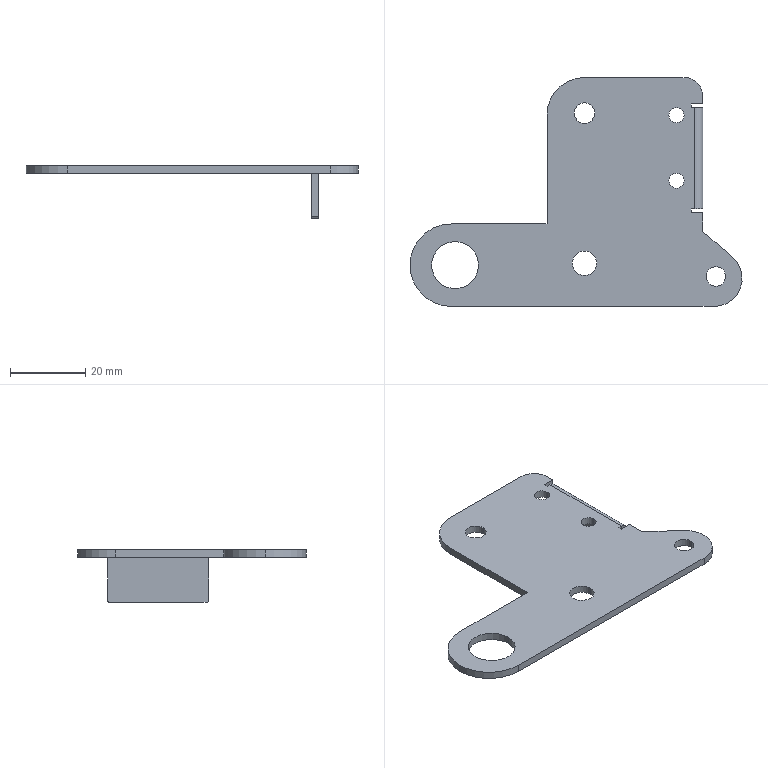Component | SolidWorks | CLS-MechanismLimitSwitchStopPlate-1 | 1 solid | 43 faces | volume 6967 mm3 | plane 22 | cylinder 21 | commonest cylinder face diameters 4 x4 6.5 x2 5.2 x2 5.5 x2 12.5 x2 22 x2 1 x2 15 x1 | material 2.0 Galvanized Sheet Q235A